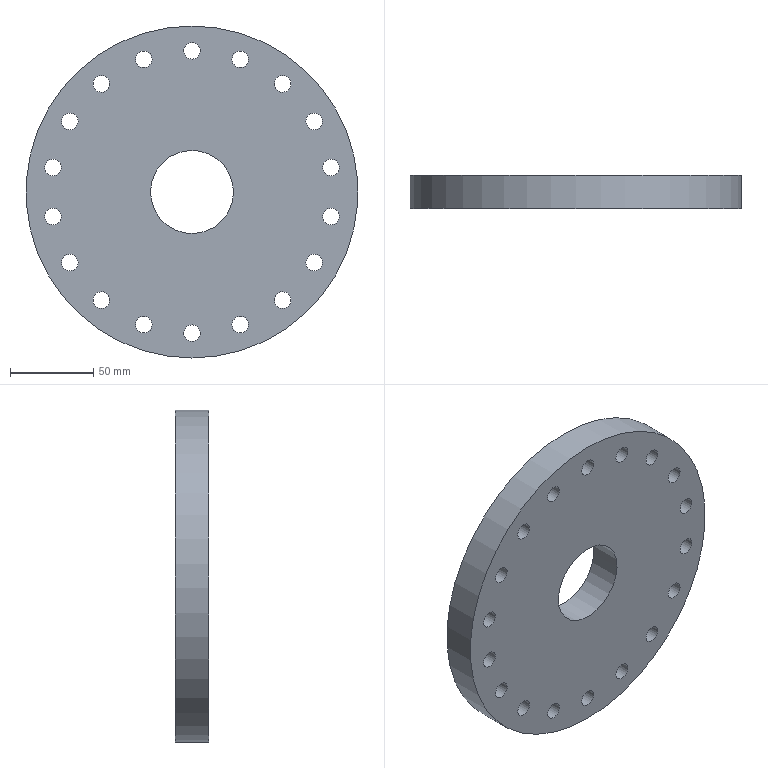Component | NX | CARK3 | 1 solid | 22 faces | volume 560774 mm3 | cylinder 20 | plane 2 | commonest cylinder face diameters 10 x18 50 x1 200 x1